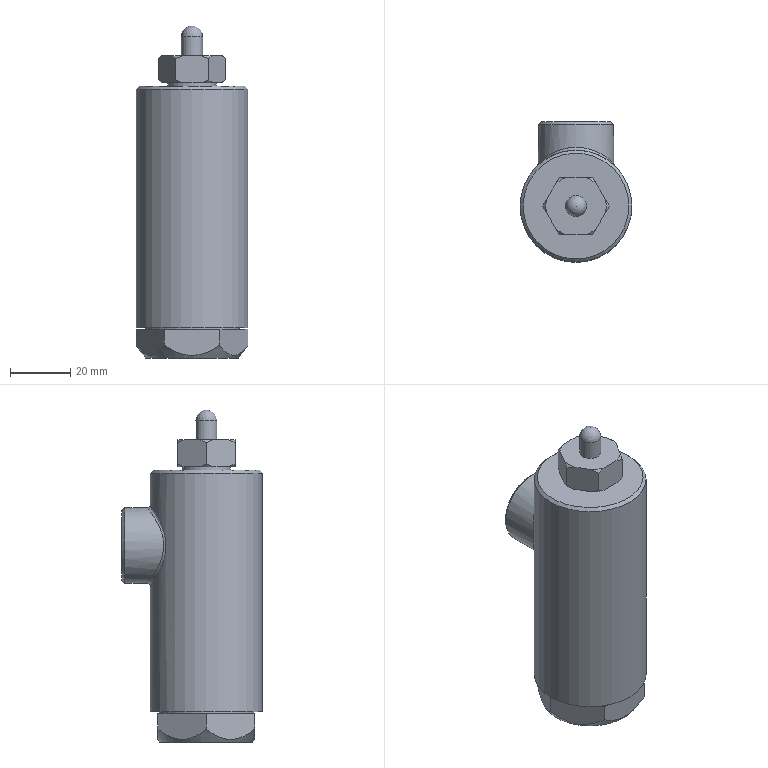Assembly | NX | mm | 7 component files | 7 solids | 96 faces | box 37 x 46.5 x 109.86 mm | volume 83146 mm3 | plane 44 | cone 24 | cylinder 21 | spline 6 | sphere 1 | commonest cylinder face diameters 7 x5 16 x3 10.3 x2 22.5 x2 37 x1 25 x1 20 x1 12 x1
Bill of materials:
GB93-87,24 | 1 |  | Single Coil Spring Lock Washer, Normal Type, GB 93-87,24
unnamed part 1 | 1 |  | Hexagonal prism base with a coaxial cylindrical boss on one face and a central axial through-hole; hex outer corners chamfered on the end away from the boss.
unnamed part 2 | 1 |  | Hexagonal head with chamfered corners on both ends, a coaxial plain cylindrical shank and a central axial through-bore.
unnamed part 3 | 1 |  | Cylindrical body with an axial through-bore and a short cylindrical side boss set perpendicular to the main axis; the boss has a hole with a chamfered or countersunk entry.
unnamed part 4 | 1 |  | Thick-walled cylindrical ring or sleeve with a large central through-bore and a 45-degree-like chamfer on the outer edge at one end.
unnamed part 5 | 1 |  | Open-coil helical spring made from round wire, roughly a dozen coils, with flattened or closed end coils.
unnamed part 6 | 1 |  | Slender cylindrical pin with a rounded (domed) tip on its long end and a thin circular flange near the other end, below which a short stub extends.
Mates:
1. fix | Valve_Body 1 component
2. touch align | Gasket 1 | Valve_Body 1 face
3. touch align | Gasket 1 | Valve_Body 1 face
4. touch align | Spring 1 | Valve_Stem 1
5. fix | Valve_Stem 1 component
6. touch align | Valve_Stem 1 | Spring 1 datumaxis